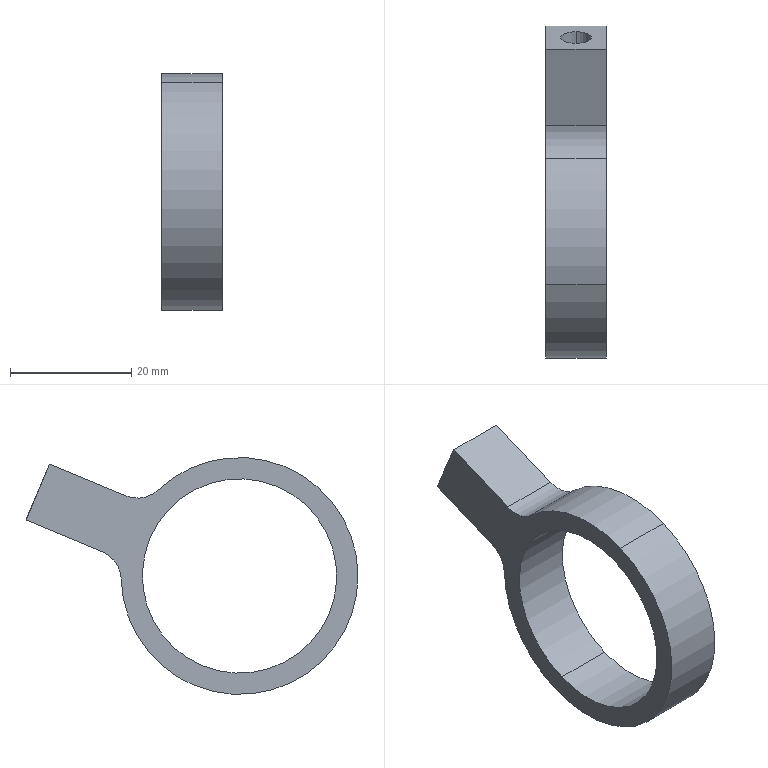Component | SolidWorks | ConnectingRod-1 | 1 solid | 16 faces | box 10 x 54.66 x 39 mm | volume 5293 mm3 | cylinder 9 | plane 5 | cone 2 | commonest cylinder face diameters 39 x3 5 x2 32 x2 10 x2 | material 6061 Alloy
build123d program:
from build123d import *

# Parameters (mm, degrees)
SKETCH1_R             = 19.5
SKETCH1_R_2           = 16
BOSS_EXTRUDE1_DEPTH   = 5
SKETCH2_W             = 18.107
SKETCH2_H             = 10
BOSS_EXTRUDE2_DEPTH   = 10
FILLET1_R             = 5
M6_TAPPED_HOLE1_D     = 5
M6_TAPPED_HOLE1_DEPTH = 16
M6_TAPPED_HOLE1_TIP   = 1.502


with BuildPart() as part:
    # Sketch1 → Boss-Extrude1 (new, symmetric)
    with BuildSketch(Plane(origin=(0, 0, 0), x_dir=(1, 0, 0), z_dir=(0, 1, 0))):
        with Locations(Location((0, 0, 0), (0, 0, 270))):
            Circle(SKETCH1_R)
        with Locations(Location((0, 0, 0), (0, 0, 270))):
            Circle(SKETCH1_R_2, mode=Mode.SUBTRACT)
    extrude(amount=BOSS_EXTRUDE1_DEPTH, both=True)

    # Sketch2 → Boss-Extrude2 (add)
    with BuildSketch(Plane(origin=(0, 5, 0), x_dir=(1, 0, 0), z_dir=(0, 1, 0))):
        with Locations((26.947, 0)):
            Rectangle(SKETCH2_W, SKETCH2_H)
    extrude(amount=-BOSS_EXTRUDE2_DEPTH)

    # Fillet1
    fillet1_edges = [part.edges().sort_by_distance(p)[0] for p in [
        (18.848, 0, 5),
        (18.848, 0, -5),
    ]]
    fillet(fillet1_edges, radius=FILLET1_R)

    # M6 Tapped Hole1
    with Locations(Plane(origin=(36, 0, 0), x_dir=(0, 0, -1), z_dir=(1, 0, 0))):
        with Locations((0, 0)):
            Hole(M6_TAPPED_HOLE1_D / 2, depth=M6_TAPPED_HOLE1_DEPTH)
            with Locations((0, 0, -(M6_TAPPED_HOLE1_DEPTH + M6_TAPPED_HOLE1_TIP / 2))):  # 118° drill point
                Cone(0, M6_TAPPED_HOLE1_D / 2, M6_TAPPED_HOLE1_TIP, mode=Mode.SUBTRACT)


solid = part.part

# Placed as in the assembly
solid = solid.moved(Location((5.226, -5.409, 81.863), (22.584, 0, 90)))
STEP:
#1=COLOUR_RGB('',0.7922,0.8196,0.9333);
#2=FILL_AREA_STYLE_COLOUR('',#1);
#3=FILL_AREA_STYLE('',(#2));
#4=SURFACE_STYLE_FILL_AREA(#3);
#5=SURFACE_SIDE_STYLE('',(#4));
#6=SURFACE_STYLE_USAGE(.BOTH.,#5);
#7=PRESENTATION_STYLE_ASSIGNMENT((#6));
#8=CARTESIAN_POINT('',(0.2058,0.4763,3.616));
#9=VERTEX_POINT('',#8);
#10=CARTESIAN_POINT('',(0.2058,0.5519,3.434));
#11=VERTEX_POINT('',#10);
#12=CARTESIAN_POINT('',(0.2058,0.5141,3.525));
#13=DIRECTION('',(0.,0.9233,0.384));
#14=DIRECTION('',(0.,0.384,-0.9233));
#15=AXIS2_PLACEMENT_3D('',#12,#13,#14);
#16=CIRCLE('',#15,0.09843);
#17=EDGE_CURVE('',#9,#11,#16,.T.);
#18=ORIENTED_EDGE('',*,*,#17,.F.);
#19=CARTESIAN_POINT('',(0.2058,1.058,3.858));
#20=VERTEX_POINT('',#19);
#21=CARTESIAN_POINT('',(0.2058,1.058,3.858));
#22=DIRECTION('',(0.,0.9233,0.384));
#23=VECTOR('',#22,39.37);
#24=LINE('',#21,#23);
#25=EDGE_CURVE('',#9,#20,#24,.T.);
#26=ORIENTED_EDGE('',*,*,#25,.T.);
#27=CARTESIAN_POINT('',(0.2058,1.133,3.676));
#28=VERTEX_POINT('',#27);
#29=CARTESIAN_POINT('',(0.2058,1.096,3.767));
#30=DIRECTION('',(0.,0.9233,0.384));
#31=DIRECTION('',(0.,0.384,-0.9233));
#32=AXIS2_PLACEMENT_3D('',#29,#30,#31);
#33=CIRCLE('',#32,0.09843);
#34=EDGE_CURVE('',#20,#28,#33,.T.);
#35=ORIENTED_EDGE('',*,*,#34,.T.);
#36=CARTESIAN_POINT('',(0.2058,1.133,3.676));
#37=DIRECTION('',(0.,0.9233,0.384));
#38=VECTOR('',#37,39.37);
#39=LINE('',#36,#38);
#40=EDGE_CURVE('',#11,#28,#39,.T.);
#41=ORIENTED_EDGE('',*,*,#40,.F.);
#42=EDGE_LOOP('',(#18,#26,#35,#41));
#43=FACE_OUTER_BOUND('',#42,.T.);
#44=CARTESIAN_POINT('',(0.2058,1.096,3.767));
#45=DIRECTION('',(0.,0.9233,0.384));
#46=DIRECTION('',(0.,0.384,-0.9233));
#47=AXIS2_PLACEMENT_3D('',#44,#45,#46);
#48=CYLINDRICAL_SURFACE('',#47,0.09843);
#49=ADVANCED_FACE('',(#43),#48,.F.);
#50=CARTESIAN_POINT('',(0.2058,0.4594,3.503));
#51=VERTEX_POINT('',#50);
#52=CARTESIAN_POINT('',(0.2058,0.5519,3.434));
#53=DIRECTION('',(0.,0.8047,-0.5936));
#54=VECTOR('',#53,39.37);
#55=LINE('',#52,#54);
#56=EDGE_CURVE('',#51,#11,#55,.T.);
#57=ORIENTED_EDGE('',*,*,#56,.F.);
#58=CARTESIAN_POINT('',(0.2058,0.4763,3.616));
#59=DIRECTION('',(0.,0.1464,0.9892));
#60=VECTOR('',#59,39.37);
#61=LINE('',#58,#60);
#62=EDGE_CURVE('',#51,#9,#61,.T.);
#63=ORIENTED_EDGE('',*,*,#62,.T.);
#64=ORIENTED_EDGE('',*,*,#17,.T.);
#65=EDGE_LOOP('',(#57,#63,#64));
#66=FACE_OUTER_BOUND('',#65,.T.);
#67=CARTESIAN_POINT('',(0.2058,0.5141,3.525));
#68=DIRECTION('',(0.,0.9233,0.384));
#69=DIRECTION('',(0.,0.384,-0.9233));
#70=AXIS2_PLACEMENT_3D('',#67,#68,#69);
#71=CONICAL_SURFACE('',#70,0.09843,1.03);
#72=ADVANCED_FACE('',(#66),#71,.F.);
#73=CARTESIAN_POINT('',(0.008912,0.02895,2.641));
#74=VERTEX_POINT('',#73);
#75=CARTESIAN_POINT('',(0.008912,-0.4549,3.805));
#76=VERTEX_POINT('',#75);
#77=CARTESIAN_POINT('',(0.008912,-0.213,3.223));
#78=DIRECTION('',(-1.,0.,0.));
#79=DIRECTION('',(0.,-0.384,0.9233));
#80=AXIS2_PLACEMENT_3D('',#77,#78,#79);
#81=CIRCLE('',#80,0.6299);
#82=EDGE_CURVE('',#74,#76,#81,.T.);
#83=ORIENTED_EDGE('',*,*,#82,.T.);
#84=CARTESIAN_POINT('',(0.4026,-0.4549,3.805));
#85=VERTEX_POINT('',#84);
#86=CARTESIAN_POINT('',(0.008912,-0.4549,3.805));
#87=DIRECTION('',(1.,-0.,-0.));
#88=VECTOR('',#87,39.37);
#89=LINE('',#86,#88);
#90=EDGE_CURVE('',#76,#85,#89,.T.);
#91=ORIENTED_EDGE('',*,*,#90,.T.);
#92=CARTESIAN_POINT('',(0.4026,0.02895,2.641));
#93=VERTEX_POINT('',#92);
#94=CARTESIAN_POINT('',(0.4026,-0.213,3.223));
#95=DIRECTION('',(-1.,0.,0.));
#96=DIRECTION('',(0.,-0.384,0.9233));
#97=AXIS2_PLACEMENT_3D('',#94,#95,#96);
#98=CIRCLE('',#97,0.6299);
#99=EDGE_CURVE('',#93,#85,#98,.T.);
#100=ORIENTED_EDGE('',*,*,#99,.F.);
#101=CARTESIAN_POINT('',(0.008912,0.02895,2.641));
#102=DIRECTION('',(1.,-0.,-0.));
#103=VECTOR('',#102,39.37);
#104=LINE('',#101,#103);
#105=EDGE_CURVE('',#74,#93,#104,.T.);
#106=ORIENTED_EDGE('',*,*,#105,.F.);
#107=EDGE_LOOP('',(#83,#91,#100,#106));
#108=FACE_OUTER_BOUND('',#107,.T.);
#109=CARTESIAN_POINT('',(0.008912,-0.213,3.223));
#110=DIRECTION('',(1.,-0.,-0.));
#111=DIRECTION('',(-0.,0.384,-0.9233));
#112=AXIS2_PLACEMENT_3D('',#109,#110,#111);
#113=CYLINDRICAL_SURFACE('',#112,0.6299);
#114=ADVANCED_FACE('',(#108),#113,.F.);
#115=CARTESIAN_POINT('',(0.008912,-0.5078,3.932));
#116=VERTEX_POINT('',#115);
#117=CARTESIAN_POINT('',(0.008912,0.3138,3.781));
#118=VERTEX_POINT('',#117);
#119=CARTESIAN_POINT('',(0.008912,-0.213,3.223));
#120=DIRECTION('',(-1.,0.,0.));
#121=DIRECTION('',(0.,-0.384,0.9233));
#122=AXIS2_PLACEMENT_3D('',#119,#120,#121);
#123=CIRCLE('',#122,0.7677);
#124=EDGE_CURVE('',#116,#118,#123,.T.);
#125=ORIENTED_EDGE('',*,*,#124,.F.);
#126=CARTESIAN_POINT('',(0.4026,-0.5078,3.932));
#127=VERTEX_POINT('',#126);
#128=CARTESIAN_POINT('',(0.008912,-0.5078,3.932));
#129=DIRECTION('',(1.,-0.,-0.));
#130=VECTOR('',#129,39.37);
#131=LINE('',#128,#130);
#132=EDGE_CURVE('',#116,#127,#131,.T.);
#133=ORIENTED_EDGE('',*,*,#132,.T.);
#134=CARTESIAN_POINT('',(0.4026,0.3138,3.781));
#135=VERTEX_POINT('',#134);
#136=CARTESIAN_POINT('',(0.4026,-0.213,3.223));
#137=DIRECTION('',(-1.,0.,0.));
#138=DIRECTION('',(0.,-0.384,0.9233));
#139=AXIS2_PLACEMENT_3D('',#136,#137,#138);
#140=CIRCLE('',#139,0.7677);
#141=EDGE_CURVE('',#127,#135,#140,.T.);
#142=ORIENTED_EDGE('',*,*,#141,.T.);
#143=CARTESIAN_POINT('',(0.008912,0.3138,3.781));
#144=DIRECTION('',(-1.,0.,0.));
#145=VECTOR('',#144,39.37);
#146=LINE('',#143,#145);
#147=EDGE_CURVE('',#135,#118,#146,.T.);
#148=ORIENTED_EDGE('',*,*,#147,.T.);
#149=EDGE_LOOP('',(#125,#133,#142,#148));
#150=FACE_OUTER_BOUND('',#149,.T.);
#151=CARTESIAN_POINT('',(0.008912,-0.213,3.223));
#152=DIRECTION('',(1.,-0.,-0.));
#153=DIRECTION('',(-0.,0.384,-0.9233));
#154=AXIS2_PLACEMENT_3D('',#151,#152,#153);
#155=CYLINDRICAL_SURFACE('',#154,0.7677);
#156=ADVANCED_FACE('',(#150),#155,.T.);
#157=ORIENTED_EDGE('',*,*,#132,.F.);
#158=CARTESIAN_POINT('',(0.008912,0.08186,2.514));
#159=VERTEX_POINT('',#158);
#160=CARTESIAN_POINT('',(0.008912,-0.213,3.223));
#161=DIRECTION('',(-1.,0.,0.));
#162=DIRECTION('',(0.,-0.384,0.9233));
#163=AXIS2_PLACEMENT_3D('',#160,#161,#162);
#164=CIRCLE('',#163,0.7677);
#165=EDGE_CURVE('',#159,#116,#164,.T.);
#166=ORIENTED_EDGE('',*,*,#165,.F.);
#167=CARTESIAN_POINT('',(0.4026,0.08186,2.514));
#168=VERTEX_POINT('',#167);
#169=CARTESIAN_POINT('',(0.008912,0.08186,2.514));
#170=DIRECTION('',(1.,-0.,-0.));
#171=VECTOR('',#170,39.37);
#172=LINE('',#169,#171);
#173=EDGE_CURVE('',#159,#168,#172,.T.);
#174=ORIENTED_EDGE('',*,*,#173,.T.);
#175=CARTESIAN_POINT('',(0.4026,-0.213,3.223));
#176=DIRECTION('',(-1.,0.,0.));
#177=DIRECTION('',(0.,-0.384,0.9233));
#178=AXIS2_PLACEMENT_3D('',#175,#176,#177);
#179=CIRCLE('',#178,0.7677);
#180=EDGE_CURVE('',#168,#127,#179,.T.);
#181=ORIENTED_EDGE('',*,*,#180,.T.);
#182=EDGE_LOOP('',(#157,#166,#174,#181));
#183=FACE_OUTER_BOUND('',#182,.T.);
#184=CARTESIAN_POINT('',(0.008912,-0.213,3.223));
#185=DIRECTION('',(1.,-0.,-0.));
#186=DIRECTION('',(-0.,0.384,-0.9233));
#187=AXIS2_PLACEMENT_3D('',#184,#185,#186);
#188=CYLINDRICAL_SURFACE('',#187,0.7677);
#189=ADVANCED_FACE('',(#183),#188,.T.);
#190=CARTESIAN_POINT('',(0.008912,1.171,3.585));
#191=VERTEX_POINT('',#190);
#192=CARTESIAN_POINT('',(0.008912,0.6757,3.379));
#193=VERTEX_POINT('',#192);
#194=CARTESIAN_POINT('',(0.008912,1.171,3.585));
#195=DIRECTION('',(-0.,-0.9233,-0.384));
#196=VECTOR('',#195,39.37);
#197=LINE('',#194,#196);
#198=EDGE_CURVE('',#191,#193,#197,.T.);
#199=ORIENTED_EDGE('',*,*,#198,.T.);
#200=CARTESIAN_POINT('',(0.008912,0.5545,3.203));
#201=VERTEX_POINT('',#200);
#202=CARTESIAN_POINT('',(0.008912,0.7513,3.198));
#203=DIRECTION('',(1.,-0.,-0.));
#204=DIRECTION('',(0.,-0.384,0.9233));
#205=AXIS2_PLACEMENT_3D('',#202,#203,#204);
#206=CIRCLE('',#205,0.1969);
#207=EDGE_CURVE('',#193,#201,#206,.T.);
#208=ORIENTED_EDGE('',*,*,#207,.T.);
#209=CARTESIAN_POINT('',(0.008912,-0.213,3.223));
#210=DIRECTION('',(-1.,0.,0.));
#211=DIRECTION('',(0.,-0.384,0.9233));
#212=AXIS2_PLACEMENT_3D('',#209,#210,#211);
#213=CIRCLE('',#212,0.7677);
#214=EDGE_CURVE('',#201,#159,#213,.T.);
#215=ORIENTED_EDGE('',*,*,#214,.T.);
#216=ORIENTED_EDGE('',*,*,#165,.T.);
#217=ORIENTED_EDGE('',*,*,#124,.T.);
#218=CARTESIAN_POINT('',(0.008912,0.5245,3.743));
#219=VERTEX_POINT('',#218);
#220=CARTESIAN_POINT('',(0.008912,0.4489,3.925));
#221=DIRECTION('',(1.,-0.,-0.));
#222=DIRECTION('',(0.,-0.384,0.9233));
#223=AXIS2_PLACEMENT_3D('',#220,#221,#222);
#224=CIRCLE('',#223,0.1969);
#225=EDGE_CURVE('',#118,#219,#224,.T.);
#226=ORIENTED_EDGE('',*,*,#225,.T.);
#227=CARTESIAN_POINT('',(0.008912,1.02,3.949));
#228=VERTEX_POINT('',#227);
#229=CARTESIAN_POINT('',(0.008912,1.02,3.949));
#230=DIRECTION('',(0.,0.9233,0.384));
#231=VECTOR('',#230,39.37);
#232=LINE('',#229,#231);
#233=EDGE_CURVE('',#219,#228,#232,.T.);
#234=ORIENTED_EDGE('',*,*,#233,.T.);
#235=CARTESIAN_POINT('',(0.008912,1.171,3.585));
#236=DIRECTION('',(-0.,0.384,-0.9233));
#237=VECTOR('',#236,39.37);
#238=LINE('',#235,#237);
#239=EDGE_CURVE('',#228,#191,#238,.T.);
#240=ORIENTED_EDGE('',*,*,#239,.T.);
#241=EDGE_LOOP('',(#199,#208,#215,#216,#217,#226,#234,#240));
#242=FACE_OUTER_BOUND('',#241,.T.);
#243=ORIENTED_EDGE('',*,*,#82,.F.);
#244=CARTESIAN_POINT('',(0.008912,-0.213,3.223));
#245=DIRECTION('',(-1.,0.,0.));
#246=DIRECTION('',(0.,-0.384,0.9233));
#247=AXIS2_PLACEMENT_3D('',#244,#245,#246);
#248=CIRCLE('',#247,0.6299);
#249=EDGE_CURVE('',#76,#74,#248,.T.);
#250=ORIENTED_EDGE('',*,*,#249,.F.);
#251=EDGE_LOOP('',(#243,#250));
#252=FACE_BOUND('',#251,.T.);
#253=CARTESIAN_POINT('',(0.008912,-0.213,3.223));
#254=DIRECTION('',(-1.,0.,0.));
#255=DIRECTION('',(0.,-0.384,0.9233));
#256=AXIS2_PLACEMENT_3D('',#253,#254,#255);
#257=PLANE('',#256);
#258=ADVANCED_FACE('',(#242,#252),#257,.T.);
#259=CARTESIAN_POINT('',(0.4026,0.5545,3.203));
#260=VERTEX_POINT('',#259);
#261=CARTESIAN_POINT('',(0.4026,-0.213,3.223));
#262=DIRECTION('',(-1.,0.,0.));
#263=DIRECTION('',(0.,-0.384,0.9233));
#264=AXIS2_PLACEMENT_3D('',#261,#262,#263);
#265=CIRCLE('',#264,0.7677);
#266=EDGE_CURVE('',#260,#168,#265,.T.);
#267=ORIENTED_EDGE('',*,*,#266,.F.);
#268=CARTESIAN_POINT('',(0.4026,0.6757,3.379));
#269=VERTEX_POINT('',#268);
#270=CARTESIAN_POINT('',(0.4026,0.7513,3.198));
#271=DIRECTION('',(-1.,0.,0.));
#272=DIRECTION('',(0.,-0.384,0.9233));
#273=AXIS2_PLACEMENT_3D('',#270,#271,#272);
#274=CIRCLE('',#273,0.1969);
#275=EDGE_CURVE('',#260,#269,#274,.T.);
#276=ORIENTED_EDGE('',*,*,#275,.T.);
#277=CARTESIAN_POINT('',(0.4026,1.171,3.585));
#278=VERTEX_POINT('',#277);
#279=CARTESIAN_POINT('',(0.4026,1.171,3.585));
#280=DIRECTION('',(0.,0.9233,0.384));
#281=VECTOR('',#280,39.37);
#282=LINE('',#279,#281);
#283=EDGE_CURVE('',#269,#278,#282,.T.);
#284=ORIENTED_EDGE('',*,*,#283,.T.);
#285=CARTESIAN_POINT('',(0.4026,1.02,3.949));
#286=VERTEX_POINT('',#285);
#287=CARTESIAN_POINT('',(0.4026,1.171,3.585));
#288=DIRECTION('',(0.,-0.384,0.9233));
#289=VECTOR('',#288,39.37);
#290=LINE('',#287,#289);
#291=EDGE_CURVE('',#278,#286,#290,.T.);
#292=ORIENTED_EDGE('',*,*,#291,.T.);
#293=CARTESIAN_POINT('',(0.4026,0.5245,3.743));
#294=VERTEX_POINT('',#293);
#295=CARTESIAN_POINT('',(0.4026,1.02,3.949));
#296=DIRECTION('',(-0.,-0.9233,-0.384));
#297=VECTOR('',#296,39.37);
#298=LINE('',#295,#297);
#299=EDGE_CURVE('',#286,#294,#298,.T.);
#300=ORIENTED_EDGE('',*,*,#299,.T.);
#301=CARTESIAN_POINT('',(0.4026,0.4489,3.925));
#302=DIRECTION('',(-1.,0.,0.));
#303=DIRECTION('',(0.,-0.384,0.9233));
#304=AXIS2_PLACEMENT_3D('',#301,#302,#303);
#305=CIRCLE('',#304,0.1969);
#306=EDGE_CURVE('',#294,#135,#305,.T.);
#307=ORIENTED_EDGE('',*,*,#306,.T.);
#308=ORIENTED_EDGE('',*,*,#141,.F.);
#309=ORIENTED_EDGE('',*,*,#180,.F.);
#310=EDGE_LOOP('',(#267,#276,#284,#292,#300,#307,#308,#309));
#311=FACE_OUTER_BOUND('',#310,.T.);
#312=ORIENTED_EDGE('',*,*,#99,.T.);
#313=CARTESIAN_POINT('',(0.4026,-0.213,3.223));
#314=DIRECTION('',(-1.,0.,0.));
#315=DIRECTION('',(0.,-0.384,0.9233));
#316=AXIS2_PLACEMENT_3D('',#313,#314,#315);
#317=CIRCLE('',#316,0.6299);
#318=EDGE_CURVE('',#85,#93,#317,.T.);
#319=ORIENTED_EDGE('',*,*,#318,.T.);
#320=EDGE_LOOP('',(#312,#319));
#321=FACE_BOUND('',#320,.T.);
#322=CARTESIAN_POINT('',(0.4026,-0.213,3.223));
#323=DIRECTION('',(-1.,0.,0.));
#324=DIRECTION('',(0.,-0.384,0.9233));
#325=AXIS2_PLACEMENT_3D('',#322,#323,#324);
#326=PLANE('',#325);
#327=ADVANCED_FACE('',(#311,#321),#326,.F.);
#328=ORIENTED_EDGE('',*,*,#173,.F.);
#329=ORIENTED_EDGE('',*,*,#214,.F.);
#330=CARTESIAN_POINT('',(0.008912,0.5545,3.203));
#331=DIRECTION('',(1.,-0.,-0.));
#332=VECTOR('',#331,39.37);
#333=LINE('',#330,#332);
#334=EDGE_CURVE('',#201,#260,#333,.T.);
#335=ORIENTED_EDGE('',*,*,#334,.T.);
#336=ORIENTED_EDGE('',*,*,#266,.T.);
#337=EDGE_LOOP('',(#328,#329,#335,#336));
#338=FACE_OUTER_BOUND('',#337,.T.);
#339=CARTESIAN_POINT('',(0.008912,-0.213,3.223));
#340=DIRECTION('',(1.,-0.,-0.));
#341=DIRECTION('',(-0.,0.384,-0.9233));
#342=AXIS2_PLACEMENT_3D('',#339,#340,#341);
#343=CYLINDRICAL_SURFACE('',#342,0.7677);
#344=ADVANCED_FACE('',(#338),#343,.T.);
#345=ORIENTED_EDGE('',*,*,#90,.F.);
#346=ORIENTED_EDGE('',*,*,#249,.T.);
#347=ORIENTED_EDGE('',*,*,#105,.T.);
#348=ORIENTED_EDGE('',*,*,#318,.F.);
#349=EDGE_LOOP('',(#345,#346,#347,#348));
#350=FACE_OUTER_BOUND('',#349,.T.);
#351=CARTESIAN_POINT('',(0.008912,-0.213,3.223));
#352=DIRECTION('',(1.,-0.,-0.));
#353=DIRECTION('',(-0.,0.384,-0.9233));
#354=AXIS2_PLACEMENT_3D('',#351,#352,#353);
#355=CYLINDRICAL_SURFACE('',#354,0.6299);
#356=ADVANCED_FACE('',(#350),#355,.F.);
#357=ORIENTED_EDGE('',*,*,#283,.F.);
#358=CARTESIAN_POINT('',(1.217,0.6757,3.379));
#359=DIRECTION('',(-1.,0.,0.));
#360=VECTOR('',#359,39.37);
#361=LINE('',#358,#360);
#362=EDGE_CURVE('',#269,#193,#361,.T.);
#363=ORIENTED_EDGE('',*,*,#362,.T.);
#364=ORIENTED_EDGE('',*,*,#198,.F.);
#365=CARTESIAN_POINT('',(1.217,1.171,3.585));
#366=DIRECTION('',(-1.,0.,0.));
#367=VECTOR('',#366,39.37);
#368=LINE('',#365,#367);
#369=EDGE_CURVE('',#278,#191,#368,.T.);
#370=ORIENTED_EDGE('',*,*,#369,.F.);
#371=EDGE_LOOP('',(#357,#363,#364,#370));
#372=FACE_OUTER_BOUND('',#371,.T.);
#373=CARTESIAN_POINT('',(1.217,1.171,3.585));
#374=DIRECTION('',(-0.,0.384,-0.9233));
#375=DIRECTION('',(-0.,-0.9233,-0.384));
#376=AXIS2_PLACEMENT_3D('',#373,#374,#375);
#377=PLANE('',#376);
#378=ADVANCED_FACE('',(#372),#377,.T.);
#379=ORIENTED_EDGE('',*,*,#233,.F.);
#380=CARTESIAN_POINT('',(1.217,0.5245,3.743));
#381=DIRECTION('',(1.,-0.,-0.));
#382=VECTOR('',#381,39.37);
#383=LINE('',#380,#382);
#384=EDGE_CURVE('',#219,#294,#383,.T.);
#385=ORIENTED_EDGE('',*,*,#384,.T.);
#386=ORIENTED_EDGE('',*,*,#299,.F.);
#387=CARTESIAN_POINT('',(1.217,1.02,3.949));
#388=DIRECTION('',(-1.,0.,0.));
#389=VECTOR('',#388,39.37);
#390=LINE('',#387,#389);
#391=EDGE_CURVE('',#286,#228,#390,.T.);
#392=ORIENTED_EDGE('',*,*,#391,.T.);
#393=EDGE_LOOP('',(#379,#385,#386,#392));
#394=FACE_OUTER_BOUND('',#393,.T.);
#395=CARTESIAN_POINT('',(1.217,1.02,3.949));
#396=DIRECTION('',(0.,-0.384,0.9233));
#397=DIRECTION('',(0.,0.9233,0.384));
#398=AXIS2_PLACEMENT_3D('',#395,#396,#397);
#399=PLANE('',#398);
#400=ADVANCED_FACE('',(#394),#399,.T.);
#401=CARTESIAN_POINT('',(0.2058,1.096,3.767));
#402=DIRECTION('',(0.,0.9233,0.384));
#403=DIRECTION('',(0.,0.384,-0.9233));
#404=AXIS2_PLACEMENT_3D('',#401,#402,#403);
#405=CIRCLE('',#404,0.09843);
#406=EDGE_CURVE('',#28,#20,#405,.T.);
#407=ORIENTED_EDGE('',*,*,#406,.F.);
#408=ORIENTED_EDGE('',*,*,#34,.F.);
#409=EDGE_LOOP('',(#407,#408));
#410=FACE_BOUND('',#409,.T.);
#411=ORIENTED_EDGE('',*,*,#291,.F.);
#412=ORIENTED_EDGE('',*,*,#369,.T.);
#413=ORIENTED_EDGE('',*,*,#239,.F.);
#414=ORIENTED_EDGE('',*,*,#391,.F.);
#415=EDGE_LOOP('',(#411,#412,#413,#414));
#416=FACE_OUTER_BOUND('',#415,.T.);
#417=CARTESIAN_POINT('',(1.217,1.171,3.585));
#418=DIRECTION('',(0.,0.9233,0.384));
#419=DIRECTION('',(-0.,0.384,-0.9233));
#420=AXIS2_PLACEMENT_3D('',#417,#418,#419);
#421=PLANE('',#420);
#422=ADVANCED_FACE('',(#410,#416),#421,.T.);
#423=ORIENTED_EDGE('',*,*,#207,.F.);
#424=ORIENTED_EDGE('',*,*,#362,.F.);
#425=ORIENTED_EDGE('',*,*,#275,.F.);
#426=ORIENTED_EDGE('',*,*,#334,.F.);
#427=EDGE_LOOP('',(#423,#424,#425,#426));
#428=FACE_OUTER_BOUND('',#427,.T.);
#429=CARTESIAN_POINT('',(0.008912,0.7513,3.198));
#430=DIRECTION('',(1.,-0.,-0.));
#431=DIRECTION('',(-0.,0.384,-0.9233));
#432=AXIS2_PLACEMENT_3D('',#429,#430,#431);
#433=CYLINDRICAL_SURFACE('',#432,0.1969);
#434=ADVANCED_FACE('',(#428),#433,.F.);
#435=ORIENTED_EDGE('',*,*,#306,.F.);
#436=ORIENTED_EDGE('',*,*,#384,.F.);
#437=ORIENTED_EDGE('',*,*,#225,.F.);
#438=ORIENTED_EDGE('',*,*,#147,.F.);
#439=EDGE_LOOP('',(#435,#436,#437,#438));
#440=FACE_OUTER_BOUND('',#439,.T.);
#441=CARTESIAN_POINT('',(0.008912,0.4489,3.925));
#442=DIRECTION('',(1.,-0.,-0.));
#443=DIRECTION('',(-0.,0.384,-0.9233));
#444=AXIS2_PLACEMENT_3D('',#441,#442,#443);
#445=CYLINDRICAL_SURFACE('',#444,0.1969);
#446=ADVANCED_FACE('',(#440),#445,.F.);
#447=ORIENTED_EDGE('',*,*,#62,.F.);
#448=ORIENTED_EDGE('',*,*,#56,.T.);
#449=CARTESIAN_POINT('',(0.2058,0.5141,3.525));
#450=DIRECTION('',(0.,0.9233,0.384));
#451=DIRECTION('',(0.,0.384,-0.9233));
#452=AXIS2_PLACEMENT_3D('',#449,#450,#451);
#453=CIRCLE('',#452,0.09843);
#454=EDGE_CURVE('',#11,#9,#453,.T.);
#455=ORIENTED_EDGE('',*,*,#454,.T.);
#456=EDGE_LOOP('',(#447,#448,#455));
#457=FACE_OUTER_BOUND('',#456,.T.);
#458=CARTESIAN_POINT('',(0.2058,0.5141,3.525));
#459=DIRECTION('',(0.,0.9233,0.384));
#460=DIRECTION('',(0.,0.384,-0.9233));
#461=AXIS2_PLACEMENT_3D('',#458,#459,#460);
#462=CONICAL_SURFACE('',#461,0.09843,1.03);
#463=ADVANCED_FACE('',(#457),#462,.F.);
#464=ORIENTED_EDGE('',*,*,#25,.F.);
#465=ORIENTED_EDGE('',*,*,#454,.F.);
#466=ORIENTED_EDGE('',*,*,#40,.T.);
#467=ORIENTED_EDGE('',*,*,#406,.T.);
#468=EDGE_LOOP('',(#464,#465,#466,#467));
#469=FACE_OUTER_BOUND('',#468,.T.);
#470=CARTESIAN_POINT('',(0.2058,1.096,3.767));
#471=DIRECTION('',(0.,0.9233,0.384));
#472=DIRECTION('',(0.,0.384,-0.9233));
#473=AXIS2_PLACEMENT_3D('',#470,#471,#472);
#474=CYLINDRICAL_SURFACE('',#473,0.09843);
#475=ADVANCED_FACE('',(#469),#474,.F.);
#476=CLOSED_SHELL('',(#49,#72,#114,#156,#189,#258,#327,#344,#356,#378,#400,#422,#434,#446,#463,#475));
#477=MANIFOLD_SOLID_BREP('',#476);
#478=STYLED_ITEM('',(#7),#477);
#479=(LENGTH_UNIT()NAMED_UNIT(*)SI_UNIT($,.METRE.));
#480=LENGTH_MEASURE_WITH_UNIT(LENGTH_MEASURE(0.0254),#479);
#481=DIMENSIONAL_EXPONENTS(1.,0.,0.,0.,0.,0.,0.);
#482=(CONVERSION_BASED_UNIT('',#480)LENGTH_UNIT()NAMED_UNIT(#481));
#483=UNCERTAINTY_MEASURE_WITH_UNIT(LENGTH_MEASURE(0.00001),#482,'','');
#484=(NAMED_UNIT(*)PLANE_ANGLE_UNIT()SI_UNIT($,.RADIAN.));
#485=(NAMED_UNIT(*)SI_UNIT($,.STERADIAN.)SOLID_ANGLE_UNIT());
#486=(GEOMETRIC_REPRESENTATION_CONTEXT(3)GLOBAL_UNCERTAINTY_ASSIGNED_CONTEXT((#483))GLOBAL_UNIT_ASSIGNED_CONTEXT((#482,#484,#485))REPRESENTATION_CONTEXT('',''));
#487=MECHANICAL_DESIGN_GEOMETRIC_PRESENTATION_REPRESENTATION('',(#478),#486);
#488=CARTESIAN_POINT('',(0.,0.,0.));
#489=DIRECTION('',(0.,0.,1.));
#490=DIRECTION('',(1.,0.,0.));
#491=AXIS2_PLACEMENT_3D('',#488,#489,#490);
#492=(LENGTH_UNIT()NAMED_UNIT(*)SI_UNIT($,.METRE.));
#493=LENGTH_MEASURE_WITH_UNIT(LENGTH_MEASURE(0.0254),#492);
#494=DIMENSIONAL_EXPONENTS(1.,0.,0.,0.,0.,0.,0.);
#495=(CONVERSION_BASED_UNIT('',#493)LENGTH_UNIT()NAMED_UNIT(#494));
#496=UNCERTAINTY_MEASURE_WITH_UNIT(LENGTH_MEASURE(0.00001),#495,'','');
#497=(NAMED_UNIT(*)PLANE_ANGLE_UNIT()SI_UNIT($,.RADIAN.));
#498=(NAMED_UNIT(*)SI_UNIT($,.STERADIAN.)SOLID_ANGLE_UNIT());
#499=(GEOMETRIC_REPRESENTATION_CONTEXT(3)GLOBAL_UNCERTAINTY_ASSIGNED_CONTEXT((#496))GLOBAL_UNIT_ASSIGNED_CONTEXT((#495,#497,#498))REPRESENTATION_CONTEXT('',''));
#500=ADVANCED_BREP_SHAPE_REPRESENTATION('',(#477,#491),#499);
#501=PRESENTATION_LAYER_ASSIGNMENT('','',(#478));